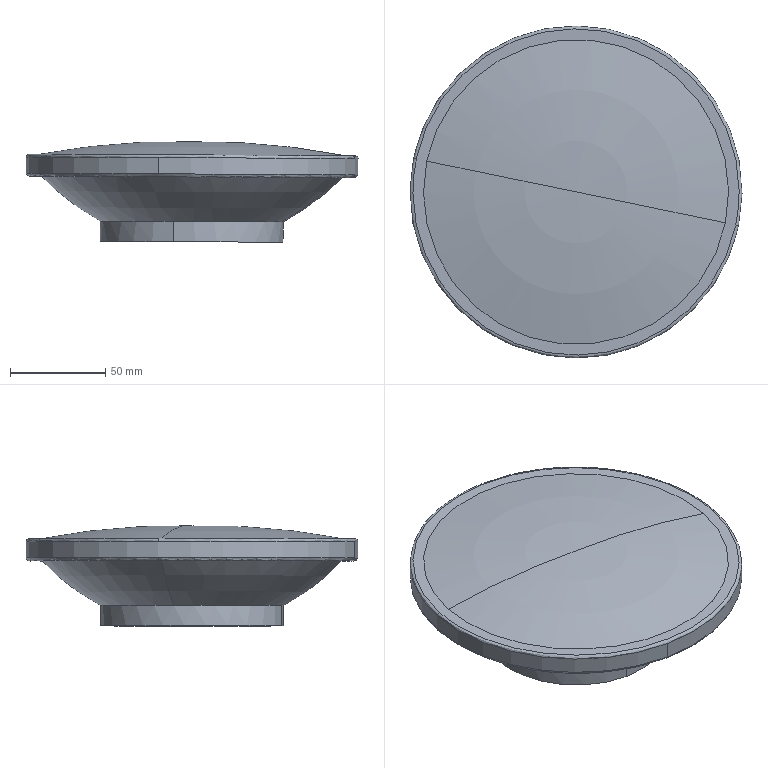Component | SolidWorks | Light-1_YellowLight-1 | 1 solid | 15 faces | box 174.03 x 174 x 52.73 mm | volume 739684 mm3 | cylinder 4 | torus 4 | spline 4 | plane 3 | commonest cylinder face diameters 96.01 x2 174 x2
STEP:
#1=COLOUR_RGB('',0.7922,0.8196,0.9333);
#2=FILL_AREA_STYLE_COLOUR('',#1);
#3=FILL_AREA_STYLE('',(#2));
#4=SURFACE_STYLE_FILL_AREA(#3);
#5=SURFACE_SIDE_STYLE('',(#4));
#6=SURFACE_STYLE_USAGE(.BOTH.,#5);
#7=PRESENTATION_STYLE_ASSIGNMENT((#6));
#8=CARTESIAN_POINT('',(-212.011,277.56,12.301));
#9=VERTEX_POINT('',#8);
#10=CARTESIAN_POINT('',(-212.776,273.859,12.304));
#11=VERTEX_POINT('',#10);
#12=CARTESIAN_POINT('',(-212.394,275.71,12.303));
#13=DIRECTION('',(-0.004294,-0.,-1.));
#14=DIRECTION('',(-0.2024,-0.9793,0.0008691));
#15=AXIS2_PLACEMENT_3D('',#12,#13,#14);
#16=CIRCLE('',#15,1.89);
#17=EDGE_CURVE('',#9,#11,#16,.T.);
#18=ORIENTED_EDGE('',*,*,#17,.F.);
#19=CARTESIAN_POINT('',(-212.009,277.56,12.72));
#20=VERTEX_POINT('',#19);
#21=CARTESIAN_POINT('',(-212.011,277.56,12.301));
#22=DIRECTION('',(0.004294,0.,1.));
#23=VECTOR('',#22,39.37);
#24=LINE('',#21,#23);
#25=EDGE_CURVE('',#9,#20,#24,.T.);
#26=ORIENTED_EDGE('',*,*,#25,.T.);
#27=CARTESIAN_POINT('',(-210.541,275.327,12.714));
#28=VERTEX_POINT('',#27);
#29=CARTESIAN_POINT('',(-212.392,275.71,12.722));
#30=DIRECTION('',(0.004294,0.,1.));
#31=DIRECTION('',(-0.9793,0.2024,0.004205));
#32=AXIS2_PLACEMENT_3D('',#29,#30,#31);
#33=CIRCLE('',#32,1.89);
#34=EDGE_CURVE('',#28,#20,#33,.T.);
#35=ORIENTED_EDGE('',*,*,#34,.F.);
#36=CARTESIAN_POINT('',(-212.774,273.859,12.724));
#37=VERTEX_POINT('',#36);
#38=CARTESIAN_POINT('',(-212.392,275.71,12.722));
#39=DIRECTION('',(0.004294,0.,1.));
#40=DIRECTION('',(-0.9793,0.2024,0.004205));
#41=AXIS2_PLACEMENT_3D('',#38,#39,#40);
#42=CIRCLE('',#41,1.89);
#43=EDGE_CURVE('',#37,#28,#42,.T.);
#44=ORIENTED_EDGE('',*,*,#43,.F.);
#45=CARTESIAN_POINT('',(-212.776,273.859,12.304));
#46=DIRECTION('',(0.004294,0.,1.));
#47=VECTOR('',#46,39.37);
#48=LINE('',#45,#47);
#49=EDGE_CURVE('',#11,#37,#48,.T.);
#50=ORIENTED_EDGE('',*,*,#49,.F.);
#51=EDGE_LOOP('',(#18,#26,#35,#44,#50));
#52=FACE_OUTER_BOUND('',#51,.T.);
#53=CARTESIAN_POINT('',(-212.394,275.71,12.303));
#54=DIRECTION('',(0.004294,0.,1.));
#55=DIRECTION('',(-0.2024,-0.9793,0.0008691));
#56=AXIS2_PLACEMENT_3D('',#53,#54,#55);
#57=CYLINDRICAL_SURFACE('',#56,1.89);
#58=ADVANCED_FACE('',(#52),#57,.T.);
#59=CARTESIAN_POINT('',(-214.243,276.092,12.73));
#60=VERTEX_POINT('',#59);
#61=CARTESIAN_POINT('',(-212.392,275.71,12.722));
#62=DIRECTION('',(0.004294,0.,1.));
#63=DIRECTION('',(-0.9793,0.2024,0.004205));
#64=AXIS2_PLACEMENT_3D('',#61,#62,#63);
#65=CIRCLE('',#64,1.89);
#66=EDGE_CURVE('',#60,#37,#65,.T.);
#67=ORIENTED_EDGE('',*,*,#66,.T.);
#68=ORIENTED_EDGE('',*,*,#43,.T.);
#69=CARTESIAN_POINT('',(-209.28,275.067,13.689));
#70=VERTEX_POINT('',#69);
#71=CARTESIAN_POINT('',(-212.982,275.836,17.344));
#72=DIRECTION('',(-0.2024,-0.9793,0.0008691));
#73=DIRECTION('',(0.9793,-0.2024,0.));
#74=AXIS2_PLACEMENT_3D('',#71,#72,#73);
#75=CIRCLE('',#74,5.259);
#76=EDGE_CURVE('',#28,#70,#75,.T.);
#77=ORIENTED_EDGE('',*,*,#76,.T.);
#78=CARTESIAN_POINT('',(-215.495,276.352,13.716));
#79=VERTEX_POINT('',#78);
#80=CARTESIAN_POINT('',(-212.388,275.71,13.702));
#81=DIRECTION('',(-0.004294,-0.,-1.));
#82=DIRECTION('',(-0.9793,0.2024,0.004205));
#83=AXIS2_PLACEMENT_3D('',#80,#81,#82);
#84=CIRCLE('',#83,3.173);
#85=EDGE_CURVE('',#70,#79,#84,.T.);
#86=ORIENTED_EDGE('',*,*,#85,.T.);
#87=CARTESIAN_POINT('',(-211.762,275.583,17.338));
#88=DIRECTION('',(0.2024,0.9793,-0.0008691));
#89=DIRECTION('',(-0.9793,0.2024,0.));
#90=AXIS2_PLACEMENT_3D('',#87,#88,#89);
#91=CIRCLE('',#90,5.259);
#92=EDGE_CURVE('',#60,#79,#91,.T.);
#93=ORIENTED_EDGE('',*,*,#92,.F.);
#94=EDGE_LOOP('',(#67,#68,#77,#86,#93));
#95=FACE_OUTER_BOUND('',#94,.T.);
#96=CARTESIAN_POINT('',(-212.372,275.71,17.341));
#97=DIRECTION('',(0.004294,0.,1.));
#98=DIRECTION('',(-0.9793,0.2024,0.004205));
#99=AXIS2_PLACEMENT_3D('',#96,#97,#98);
#100=TOROIDAL_SURFACE('',#99,-0.6233,5.259);
#101=ADVANCED_FACE('',(#95),#100,.T.);
#102=CARTESIAN_POINT('',(-211.694,279.064,13.699));
#103=VERTEX_POINT('',#102);
#104=CARTESIAN_POINT('',(-209.033,275.016,13.688));
#105=VERTEX_POINT('',#104);
#106=CARTESIAN_POINT('',(-212.388,275.71,13.702));
#107=DIRECTION('',(-0.004294,-0.,-1.));
#108=DIRECTION('',(0.9793,-0.2024,-0.004205));
#109=AXIS2_PLACEMENT_3D('',#106,#107,#108);
#110=CIRCLE('',#109,3.425);
#111=EDGE_CURVE('',#103,#105,#110,.T.);
#112=ORIENTED_EDGE('',*,*,#111,.F.);
#113=CARTESIAN_POINT('',(-211.693,279.064,14.034));
#114=VERTEX_POINT('',#113);
#115=CARTESIAN_POINT('',(-211.694,279.064,13.699));
#116=DIRECTION('',(0.004294,0.,1.));
#117=VECTOR('',#116,39.37);
#118=LINE('',#115,#117);
#119=EDGE_CURVE('',#103,#114,#118,.T.);
#120=ORIENTED_EDGE('',*,*,#119,.T.);
#121=CARTESIAN_POINT('',(-209.032,275.016,14.023));
#122=VERTEX_POINT('',#121);
#123=CARTESIAN_POINT('',(-212.386,275.71,14.037));
#124=DIRECTION('',(0.004294,0.,1.));
#125=DIRECTION('',(-0.9793,0.2024,0.004205));
#126=AXIS2_PLACEMENT_3D('',#123,#124,#125);
#127=CIRCLE('',#126,3.425);
#128=EDGE_CURVE('',#122,#114,#127,.T.);
#129=ORIENTED_EDGE('',*,*,#128,.F.);
#130=CARTESIAN_POINT('',(-213.079,272.355,14.04));
#131=VERTEX_POINT('',#130);
#132=CARTESIAN_POINT('',(-212.386,275.71,14.037));
#133=DIRECTION('',(0.004294,0.,1.));
#134=DIRECTION('',(-0.9793,0.2024,0.004205));
#135=AXIS2_PLACEMENT_3D('',#132,#133,#134);
#136=CIRCLE('',#135,3.425);
#137=EDGE_CURVE('',#131,#122,#136,.T.);
#138=ORIENTED_EDGE('',*,*,#137,.F.);
#139=CARTESIAN_POINT('',(-213.081,272.355,13.705));
#140=VERTEX_POINT('',#139);
#141=CARTESIAN_POINT('',(-213.081,272.355,13.705));
#142=DIRECTION('',(0.004294,0.,1.));
#143=VECTOR('',#142,39.37);
#144=LINE('',#141,#143);
#145=EDGE_CURVE('',#140,#131,#144,.T.);
#146=ORIENTED_EDGE('',*,*,#145,.F.);
#147=CARTESIAN_POINT('',(-212.388,275.71,13.702));
#148=DIRECTION('',(-0.004294,-0.,-1.));
#149=DIRECTION('',(-0.9793,0.2024,0.004205));
#150=AXIS2_PLACEMENT_3D('',#147,#148,#149);
#151=CIRCLE('',#150,3.425);
#152=EDGE_CURVE('',#105,#140,#151,.T.);
#153=ORIENTED_EDGE('',*,*,#152,.F.);
#154=EDGE_LOOP('',(#112,#120,#129,#138,#146,#153));
#155=FACE_OUTER_BOUND('',#154,.T.);
#156=CARTESIAN_POINT('',(-212.388,275.71,13.702));
#157=DIRECTION('',(0.004294,0.,1.));
#158=DIRECTION('',(-0.2024,-0.9793,0.0008691));
#159=AXIS2_PLACEMENT_3D('',#156,#157,#158);
#160=CYLINDRICAL_SURFACE('',#159,3.425);
#161=ADVANCED_FACE('',(#155),#160,.T.);
#162=CARTESIAN_POINT('',(-209.303,275.072,14.083));
#163=VERTEX_POINT('',#162);
#164=CARTESIAN_POINT('',(-215.469,276.347,14.109));
#165=VERTEX_POINT('',#164);
#166=CARTESIAN_POINT('',(-212.386,275.71,14.096));
#167=DIRECTION('',(-0.004294,-0.,-1.));
#168=DIRECTION('',(-0.9793,0.2024,0.004205));
#169=AXIS2_PLACEMENT_3D('',#166,#167,#168);
#170=CIRCLE('',#169,3.148);
#171=EDGE_CURVE('',#163,#165,#170,.T.);
#172=ORIENTED_EDGE('',*,*,#171,.F.);
#173=CARTESIAN_POINT('',(-212.385,275.71,14.366));
#174=VERTEX_POINT('',#173);
#175=CARTESIAN_POINT('',(-212.166,275.651,-0.7306));
#176=DIRECTION('',(-0.2024,-0.9793,0.0008691));
#177=DIRECTION('',(0.9793,-0.2024,0.));
#178=AXIS2_PLACEMENT_3D('',#175,#176,#177);
#179=CIRCLE('',#178,15.099);
#180=EDGE_CURVE('',#163,#174,#179,.T.);
#181=ORIENTED_EDGE('',*,*,#180,.T.);
#182=CARTESIAN_POINT('',(-212.733,275.768,-0.7281));
#183=DIRECTION('',(0.2024,0.9793,-0.0008691));
#184=DIRECTION('',(-0.9793,0.2024,0.));
#185=AXIS2_PLACEMENT_3D('',#182,#183,#184);
#186=CIRCLE('',#185,15.099);
#187=EDGE_CURVE('',#165,#174,#186,.T.);
#188=ORIENTED_EDGE('',*,*,#187,.F.);
#189=EDGE_LOOP('',(#172,#181,#188));
#190=FACE_OUTER_BOUND('',#189,.T.);
#191=CARTESIAN_POINT('',(-212.45,275.71,-0.7293));
#192=DIRECTION('',(0.004294,0.,1.));
#193=DIRECTION('',(-0.9793,0.2024,0.004205));
#194=AXIS2_PLACEMENT_3D('',#191,#192,#193);
#195=TOROIDAL_SURFACE('',#194,0.2891,15.099);
#196=ADVANCED_FACE('',(#190),#195,.T.);
#197=ORIENTED_EDGE('',*,*,#25,.F.);
#198=CARTESIAN_POINT('',(-212.394,275.71,12.303));
#199=DIRECTION('',(-0.004294,-0.,-1.));
#200=DIRECTION('',(-0.2024,-0.9793,0.0008691));
#201=AXIS2_PLACEMENT_3D('',#198,#199,#200);
#202=CIRCLE('',#201,1.89);
#203=EDGE_CURVE('',#11,#9,#202,.T.);
#204=ORIENTED_EDGE('',*,*,#203,.F.);
#205=ORIENTED_EDGE('',*,*,#49,.T.);
#206=ORIENTED_EDGE('',*,*,#66,.F.);
#207=CARTESIAN_POINT('',(-212.392,275.71,12.722));
#208=DIRECTION('',(0.004294,0.,1.));
#209=DIRECTION('',(-0.9793,0.2024,0.004205));
#210=AXIS2_PLACEMENT_3D('',#207,#208,#209);
#211=CIRCLE('',#210,1.89);
#212=EDGE_CURVE('',#20,#60,#211,.T.);
#213=ORIENTED_EDGE('',*,*,#212,.F.);
#214=EDGE_LOOP('',(#197,#204,#205,#206,#213));
#215=FACE_OUTER_BOUND('',#214,.T.);
#216=CARTESIAN_POINT('',(-212.394,275.71,12.303));
#217=DIRECTION('',(0.004294,0.,1.));
#218=DIRECTION('',(-0.2024,-0.9793,0.0008691));
#219=AXIS2_PLACEMENT_3D('',#216,#217,#218);
#220=CYLINDRICAL_SURFACE('',#219,1.89);
#221=ADVANCED_FACE('',(#215),#220,.T.);
#222=ORIENTED_EDGE('',*,*,#203,.T.);
#223=ORIENTED_EDGE('',*,*,#17,.T.);
#224=EDGE_LOOP('',(#222,#223));
#225=FACE_OUTER_BOUND('',#224,.T.);
#226=CARTESIAN_POINT('',(-213.879,277.97,12.309));
#227=DIRECTION('',(-0.004294,-0.,-1.));
#228=DIRECTION('',(0.9793,-0.2024,-0.004205));
#229=AXIS2_PLACEMENT_3D('',#226,#227,#228);
#230=PLANE('',#229);
#231=ADVANCED_FACE('',(#225),#230,.T.);
#232=ORIENTED_EDGE('',*,*,#76,.F.);
#233=ORIENTED_EDGE('',*,*,#34,.T.);
#234=ORIENTED_EDGE('',*,*,#212,.T.);
#235=ORIENTED_EDGE('',*,*,#92,.T.);
#236=CARTESIAN_POINT('',(-212.388,275.71,13.702));
#237=DIRECTION('',(-0.004294,-0.,-1.));
#238=DIRECTION('',(-0.9793,0.2024,0.004205));
#239=AXIS2_PLACEMENT_3D('',#236,#237,#238);
#240=CIRCLE('',#239,3.173);
#241=EDGE_CURVE('',#79,#70,#240,.T.);
#242=ORIENTED_EDGE('',*,*,#241,.T.);
#243=EDGE_LOOP('',(#232,#233,#234,#235,#242));
#244=FACE_OUTER_BOUND('',#243,.T.);
#245=CARTESIAN_POINT('',(-212.372,275.71,17.341));
#246=DIRECTION('',(0.004294,0.,1.));
#247=DIRECTION('',(-0.9793,0.2024,0.004205));
#248=AXIS2_PLACEMENT_3D('',#245,#246,#247);
#249=TOROIDAL_SURFACE('',#248,-0.6233,5.259);
#250=ADVANCED_FACE('',(#244),#249,.T.);
#251=ORIENTED_EDGE('',*,*,#241,.F.);
#252=ORIENTED_EDGE('',*,*,#85,.F.);
#253=EDGE_LOOP('',(#251,#252));
#254=FACE_BOUND('',#253,.T.);
#255=CARTESIAN_POINT('',(-209.198,275.05,13.689));
#256=VERTEX_POINT('',#255);
#257=CARTESIAN_POINT('',(-215.577,276.369,13.716));
#258=VERTEX_POINT('',#257);
#259=CARTESIAN_POINT('',(-209.198,275.05,13.689));
#260=CARTESIAN_POINT('',(-210.517,268.671,13.694));
#261=CARTESIAN_POINT('',(-216.896,269.99,13.722));
#262=CARTESIAN_POINT('',(-215.577,276.369,13.716));
#263=(BOUNDED_CURVE()B_SPLINE_CURVE(3,(#259,#260,#261,#262),.UNSPECIFIED.,.F.,.F.)B_SPLINE_CURVE_WITH_KNOTS((4,4),(0.,0.2611),.UNSPECIFIED.)CURVE()GEOMETRIC_REPRESENTATION_ITEM()RATIONAL_B_SPLINE_CURVE((0.9227,0.3076,0.3076,0.9227))REPRESENTATION_ITEM(''));
#264=EDGE_CURVE('',#256,#258,#263,.T.);
#265=ORIENTED_EDGE('',*,*,#264,.T.);
#266=CARTESIAN_POINT('',(-215.577,276.369,13.716));
#267=CARTESIAN_POINT('',(-214.259,282.748,13.71));
#268=CARTESIAN_POINT('',(-207.879,281.43,13.683));
#269=CARTESIAN_POINT('',(-209.198,275.05,13.689));
#270=(BOUNDED_CURVE()B_SPLINE_CURVE(3,(#266,#267,#268,#269),.UNSPECIFIED.,.F.,.F.)B_SPLINE_CURVE_WITH_KNOTS((4,4),(0.,0.2611),.UNSPECIFIED.)CURVE()GEOMETRIC_REPRESENTATION_ITEM()RATIONAL_B_SPLINE_CURVE((0.9227,0.3076,0.3076,0.9227))REPRESENTATION_ITEM(''));
#271=EDGE_CURVE('',#258,#256,#270,.T.);
#272=ORIENTED_EDGE('',*,*,#271,.T.);
#273=EDGE_LOOP('',(#265,#272));
#274=FACE_OUTER_BOUND('',#273,.T.);
#275=CARTESIAN_POINT('',(-214.948,279.605,13.713));
#276=DIRECTION('',(-0.004294,-0.,-1.));
#277=DIRECTION('',(0.9793,-0.2024,-0.004205));
#278=AXIS2_PLACEMENT_3D('',#275,#276,#277);
#279=PLANE('',#278);
#280=ADVANCED_FACE('',(#254,#274),#279,.T.);
#281=CARTESIAN_POINT('',(-215.742,276.403,13.717));
#282=VERTEX_POINT('',#281);
#283=CARTESIAN_POINT('',(-215.577,276.369,13.716));
#284=CARTESIAN_POINT('',(-215.606,276.375,13.61));
#285=CARTESIAN_POINT('',(-215.714,276.397,13.61));
#286=CARTESIAN_POINT('',(-215.742,276.403,13.717));
#287=(BOUNDED_CURVE()B_SPLINE_CURVE(3,(#283,#284,#285,#286),.UNSPECIFIED.,.F.,.F.)B_SPLINE_CURVE_WITH_KNOTS((4,4),(0.04868,0.9513),.UNSPECIFIED.)CURVE()GEOMETRIC_REPRESENTATION_ITEM()RATIONAL_B_SPLINE_CURVE((0.9227,0.4691,0.4691,0.9227))REPRESENTATION_ITEM(''));
#288=EDGE_CURVE('',#258,#282,#287,.T.);
#289=ORIENTED_EDGE('',*,*,#288,.T.);
#290=CARTESIAN_POINT('',(-212.388,275.71,13.702));
#291=DIRECTION('',(-0.004294,-0.,-1.));
#292=DIRECTION('',(0.9793,-0.2024,-0.004205));
#293=AXIS2_PLACEMENT_3D('',#290,#291,#292);
#294=CIRCLE('',#293,3.425);
#295=EDGE_CURVE('',#282,#103,#294,.T.);
#296=ORIENTED_EDGE('',*,*,#295,.T.);
#297=ORIENTED_EDGE('',*,*,#111,.T.);
#298=CARTESIAN_POINT('',(-209.033,275.016,13.688));
#299=CARTESIAN_POINT('',(-209.062,275.022,13.582));
#300=CARTESIAN_POINT('',(-209.17,275.044,13.582));
#301=CARTESIAN_POINT('',(-209.198,275.05,13.689));
#302=(BOUNDED_CURVE()B_SPLINE_CURVE(3,(#298,#299,#300,#301),.UNSPECIFIED.,.F.,.T.)B_SPLINE_CURVE_WITH_KNOTS((4,4),(0.04868,0.9513),.UNSPECIFIED.)CURVE()GEOMETRIC_REPRESENTATION_ITEM()RATIONAL_B_SPLINE_CURVE((0.9227,0.4691,0.4691,0.9227))REPRESENTATION_ITEM(''));
#303=EDGE_CURVE('',#105,#256,#302,.T.);
#304=ORIENTED_EDGE('',*,*,#303,.T.);
#305=ORIENTED_EDGE('',*,*,#271,.F.);
#306=EDGE_LOOP('',(#289,#296,#297,#304,#305));
#307=FACE_OUTER_BOUND('',#306,.T.);
#308=CARTESIAN_POINT('',(-209.031,275.016,13.696));
#309=CARTESIAN_POINT('',(-207.644,281.728,13.691));
#310=CARTESIAN_POINT('',(-214.356,283.116,13.719));
#311=CARTESIAN_POINT('',(-215.744,276.403,13.725));
#312=CARTESIAN_POINT('',(-209.053,275.02,13.569));
#313=CARTESIAN_POINT('',(-207.674,281.691,13.563));
#314=CARTESIAN_POINT('',(-214.344,283.069,13.592));
#315=CARTESIAN_POINT('',(-215.723,276.399,13.598));
#316=CARTESIAN_POINT('',(-209.179,275.046,13.57));
#317=CARTESIAN_POINT('',(-207.853,281.464,13.564));
#318=CARTESIAN_POINT('',(-214.27,282.79,13.592));
#319=CARTESIAN_POINT('',(-215.597,276.373,13.597));
#320=CARTESIAN_POINT('',(-209.2,275.051,13.697));
#321=CARTESIAN_POINT('',(-207.882,281.426,13.692));
#322=CARTESIAN_POINT('',(-214.257,282.744,13.719));
#323=CARTESIAN_POINT('',(-215.575,276.369,13.725));
#324=(BOUNDED_SURFACE()B_SPLINE_SURFACE(3,3,((#308,#309,#310,#311),(#312,#313,#314,#315),(#316,#317,#318,#319),(#320,#321,#322,#323)),.UNSPECIFIED.,.F.,.F.,.T.)B_SPLINE_SURFACE_WITH_KNOTS((4,4),(4,4),(0.,1.),(0.,1.),.UNSPECIFIED.)GEOMETRIC_REPRESENTATION_ITEM()RATIONAL_B_SPLINE_SURFACE(((1.,0.3333,0.3333,1.),(0.4434,0.1478,0.1478,0.4434),(0.4434,0.1478,0.1478,0.4434),(1.,0.3333,0.3333,1.)))REPRESENTATION_ITEM('')SURFACE());
#325=ADVANCED_FACE('',(#307),#324,.T.);
#326=ORIENTED_EDGE('',*,*,#152,.T.);
#327=CARTESIAN_POINT('',(-212.388,275.71,13.702));
#328=DIRECTION('',(-0.004294,-0.,-1.));
#329=DIRECTION('',(-0.9793,0.2024,0.004205));
#330=AXIS2_PLACEMENT_3D('',#327,#328,#329);
#331=CIRCLE('',#330,3.425);
#332=EDGE_CURVE('',#140,#282,#331,.T.);
#333=ORIENTED_EDGE('',*,*,#332,.T.);
#334=ORIENTED_EDGE('',*,*,#288,.F.);
#335=ORIENTED_EDGE('',*,*,#264,.F.);
#336=ORIENTED_EDGE('',*,*,#303,.F.);
#337=EDGE_LOOP('',(#326,#333,#334,#335,#336));
#338=FACE_OUTER_BOUND('',#337,.T.);
#339=CARTESIAN_POINT('',(-215.744,276.403,13.725));
#340=CARTESIAN_POINT('',(-217.131,269.691,13.731));
#341=CARTESIAN_POINT('',(-210.419,268.304,13.702));
#342=CARTESIAN_POINT('',(-209.031,275.016,13.696));
#343=CARTESIAN_POINT('',(-215.723,276.399,13.598));
#344=CARTESIAN_POINT('',(-217.102,269.729,13.604));
#345=CARTESIAN_POINT('',(-210.432,268.35,13.575));
#346=CARTESIAN_POINT('',(-209.053,275.02,13.569));
#347=CARTESIAN_POINT('',(-215.597,276.373,13.597));
#348=CARTESIAN_POINT('',(-216.923,269.955,13.603));
#349=CARTESIAN_POINT('',(-210.506,268.629,13.575));
#350=CARTESIAN_POINT('',(-209.179,275.046,13.57));
#351=CARTESIAN_POINT('',(-215.575,276.369,13.725));
#352=CARTESIAN_POINT('',(-216.893,269.993,13.73));
#353=CARTESIAN_POINT('',(-210.518,268.675,13.703));
#354=CARTESIAN_POINT('',(-209.2,275.051,13.697));
#355=(BOUNDED_SURFACE()B_SPLINE_SURFACE(3,3,((#339,#340,#341,#342),(#343,#344,#345,#346),(#347,#348,#349,#350),(#351,#352,#353,#354)),.UNSPECIFIED.,.F.,.F.,.F.)B_SPLINE_SURFACE_WITH_KNOTS((4,4),(4,4),(0.,1.),(0.,1.),.UNSPECIFIED.)GEOMETRIC_REPRESENTATION_ITEM()RATIONAL_B_SPLINE_SURFACE(((1.,0.3333,0.3333,1.),(0.4434,0.1478,0.1478,0.4434),(0.4434,0.1478,0.1478,0.4434),(1.,0.3333,0.3333,1.)))REPRESENTATION_ITEM('')SURFACE());
#356=ADVANCED_FACE('',(#338),#355,.T.);
#357=ORIENTED_EDGE('',*,*,#119,.F.);
#358=ORIENTED_EDGE('',*,*,#295,.F.);
#359=ORIENTED_EDGE('',*,*,#332,.F.);
#360=ORIENTED_EDGE('',*,*,#145,.T.);
#361=CARTESIAN_POINT('',(-215.74,276.403,14.051));
#362=VERTEX_POINT('',#361);
#363=CARTESIAN_POINT('',(-212.386,275.71,14.037));
#364=DIRECTION('',(0.004294,0.,1.));
#365=DIRECTION('',(-0.9793,0.2024,0.004205));
#366=AXIS2_PLACEMENT_3D('',#363,#364,#365);
#367=CIRCLE('',#366,3.425);
#368=EDGE_CURVE('',#362,#131,#367,.T.);
#369=ORIENTED_EDGE('',*,*,#368,.F.);
#370=CARTESIAN_POINT('',(-212.386,275.71,14.037));
#371=DIRECTION('',(0.004294,0.,1.));
#372=DIRECTION('',(-0.9793,0.2024,0.004205));
#373=AXIS2_PLACEMENT_3D('',#370,#371,#372);
#374=CIRCLE('',#373,3.425);
#375=EDGE_CURVE('',#114,#362,#374,.T.);
#376=ORIENTED_EDGE('',*,*,#375,.F.);
#377=EDGE_LOOP('',(#357,#358,#359,#360,#369,#376));
#378=FACE_OUTER_BOUND('',#377,.T.);
#379=CARTESIAN_POINT('',(-212.388,275.71,13.702));
#380=DIRECTION('',(0.004294,0.,1.));
#381=DIRECTION('',(-0.2024,-0.9793,0.0008691));
#382=AXIS2_PLACEMENT_3D('',#379,#380,#381);
#383=CYLINDRICAL_SURFACE('',#382,3.425);
#384=ADVANCED_FACE('',(#378),#383,.T.);
#385=CARTESIAN_POINT('',(-215.682,276.391,14.11));
#386=VERTEX_POINT('',#385);
#387=CARTESIAN_POINT('',(-215.74,276.403,14.051));
#388=CARTESIAN_POINT('',(-215.74,276.403,14.086));
#389=CARTESIAN_POINT('',(-215.716,276.398,14.11));
#390=CARTESIAN_POINT('',(-215.682,276.391,14.11));
#391=(BOUNDED_CURVE()B_SPLINE_CURVE(3,(#387,#388,#389,#390),.UNSPECIFIED.,.F.,.F.)B_SPLINE_CURVE_WITH_KNOTS((4,4),(0.06314,0.9369),.UNSPECIFIED.)CURVE()GEOMETRIC_REPRESENTATION_ITEM()RATIONAL_B_SPLINE_CURVE((0.9566,0.7698,0.7698,0.9566))REPRESENTATION_ITEM(''));
#392=EDGE_CURVE('',#362,#386,#391,.T.);
#393=ORIENTED_EDGE('',*,*,#392,.T.);
#394=CARTESIAN_POINT('',(-209.089,275.028,14.082));
#395=VERTEX_POINT('',#394);
#396=CARTESIAN_POINT('',(-215.682,276.391,14.11));
#397=CARTESIAN_POINT('',(-214.32,282.984,14.104));
#398=CARTESIAN_POINT('',(-207.727,281.621,14.076));
#399=CARTESIAN_POINT('',(-209.089,275.028,14.082));
#400=(BOUNDED_CURVE()B_SPLINE_CURVE(3,(#396,#397,#398,#399),.UNSPECIFIED.,.F.,.F.)B_SPLINE_CURVE_WITH_KNOTS((4,4),(0.,1.),.UNSPECIFIED.)CURVE()GEOMETRIC_REPRESENTATION_ITEM()RATIONAL_B_SPLINE_CURVE((0.9566,0.3189,0.3189,0.9566))REPRESENTATION_ITEM(''));
#401=EDGE_CURVE('',#386,#395,#400,.T.);
#402=ORIENTED_EDGE('',*,*,#401,.T.);
#403=CARTESIAN_POINT('',(-209.089,275.028,14.082));
#404=CARTESIAN_POINT('',(-209.056,275.021,14.082));
#405=CARTESIAN_POINT('',(-209.032,275.016,14.057));
#406=CARTESIAN_POINT('',(-209.032,275.016,14.023));
#407=(BOUNDED_CURVE()B_SPLINE_CURVE(3,(#403,#404,#405,#406),.UNSPECIFIED.,.F.,.T.)B_SPLINE_CURVE_WITH_KNOTS((4,4),(0.06314,0.9369),.UNSPECIFIED.)CURVE()GEOMETRIC_REPRESENTATION_ITEM()RATIONAL_B_SPLINE_CURVE((0.9566,0.7698,0.7698,0.9566))REPRESENTATION_ITEM(''));
#408=EDGE_CURVE('',#395,#122,#407,.T.);
#409=ORIENTED_EDGE('',*,*,#408,.T.);
#410=ORIENTED_EDGE('',*,*,#128,.T.);
#411=ORIENTED_EDGE('',*,*,#375,.T.);
#412=EDGE_LOOP('',(#393,#402,#409,#410,#411));
#413=FACE_OUTER_BOUND('',#412,.T.);
#414=CARTESIAN_POINT('',(-209.095,275.029,14.082));
#415=CARTESIAN_POINT('',(-207.735,281.611,14.076));
#416=CARTESIAN_POINT('',(-214.316,282.971,14.104));
#417=CARTESIAN_POINT('',(-215.677,276.39,14.11));
#418=CARTESIAN_POINT('',(-209.056,275.021,14.086));
#419=CARTESIAN_POINT('',(-207.679,281.681,14.08));
#420=CARTESIAN_POINT('',(-214.339,283.058,14.108));
#421=CARTESIAN_POINT('',(-215.716,276.398,14.114));
#422=CARTESIAN_POINT('',(-209.028,275.016,14.057));
#423=CARTESIAN_POINT('',(-207.64,281.731,14.051));
#424=CARTESIAN_POINT('',(-214.356,283.12,14.08));
#425=CARTESIAN_POINT('',(-215.744,276.404,14.086));
#426=CARTESIAN_POINT('',(-209.032,275.016,14.017));
#427=CARTESIAN_POINT('',(-207.646,281.724,14.011));
#428=CARTESIAN_POINT('',(-214.354,283.111,14.04));
#429=CARTESIAN_POINT('',(-215.74,276.403,14.046));
#430=(BOUNDED_SURFACE()B_SPLINE_SURFACE(3,3,((#414,#415,#416,#417),(#418,#419,#420,#421),(#422,#423,#424,#425),(#426,#427,#428,#429)),.UNSPECIFIED.,.F.,.F.,.F.)B_SPLINE_SURFACE_WITH_KNOTS((4,4),(4,4),(0.,1.),(0.,1.),.UNSPECIFIED.)GEOMETRIC_REPRESENTATION_ITEM()RATIONAL_B_SPLINE_SURFACE(((1.,0.3333,0.3333,1.),(0.7553,0.2518,0.2518,0.7553),(0.7553,0.2518,0.2518,0.7553),(1.,0.3333,0.3333,1.)))REPRESENTATION_ITEM('')SURFACE());
#431=ADVANCED_FACE('',(#413),#430,.T.);
#432=CARTESIAN_POINT('',(-209.089,275.028,14.082));
#433=CARTESIAN_POINT('',(-210.452,268.435,14.088));
#434=CARTESIAN_POINT('',(-217.045,269.798,14.116));
#435=CARTESIAN_POINT('',(-215.682,276.391,14.11));
#436=(BOUNDED_CURVE()B_SPLINE_CURVE(3,(#432,#433,#434,#435),.UNSPECIFIED.,.F.,.T.)B_SPLINE_CURVE_WITH_KNOTS((4,4),(0.,1.),.UNSPECIFIED.)CURVE()GEOMETRIC_REPRESENTATION_ITEM()RATIONAL_B_SPLINE_CURVE((0.9566,0.3189,0.3189,0.9566))REPRESENTATION_ITEM(''));
#437=EDGE_CURVE('',#395,#386,#436,.T.);
#438=ORIENTED_EDGE('',*,*,#437,.T.);
#439=ORIENTED_EDGE('',*,*,#392,.F.);
#440=ORIENTED_EDGE('',*,*,#368,.T.);
#441=ORIENTED_EDGE('',*,*,#137,.T.);
#442=ORIENTED_EDGE('',*,*,#408,.F.);
#443=EDGE_LOOP('',(#438,#439,#440,#441,#442));
#444=FACE_OUTER_BOUND('',#443,.T.);
#445=CARTESIAN_POINT('',(-215.677,276.39,14.11));
#446=CARTESIAN_POINT('',(-217.037,269.808,14.116));
#447=CARTESIAN_POINT('',(-210.456,268.448,14.087));
#448=CARTESIAN_POINT('',(-209.095,275.029,14.082));
#449=CARTESIAN_POINT('',(-215.716,276.398,14.114));
#450=CARTESIAN_POINT('',(-217.092,269.738,14.12));
#451=CARTESIAN_POINT('',(-210.433,268.361,14.091));
#452=CARTESIAN_POINT('',(-209.056,275.021,14.086));
#453=CARTESIAN_POINT('',(-215.744,276.404,14.086));
#454=CARTESIAN_POINT('',(-217.132,269.688,14.092));
#455=CARTESIAN_POINT('',(-210.416,268.3,14.063));
#456=CARTESIAN_POINT('',(-209.028,275.016,14.057));
#457=CARTESIAN_POINT('',(-215.74,276.403,14.046));
#458=CARTESIAN_POINT('',(-217.127,269.695,14.051));
#459=CARTESIAN_POINT('',(-210.419,268.308,14.023));
#460=CARTESIAN_POINT('',(-209.032,275.016,14.017));
#461=(BOUNDED_SURFACE()B_SPLINE_SURFACE(3,3,((#445,#446,#447,#448),(#449,#450,#451,#452),(#453,#454,#455,#456),(#457,#458,#459,#460)),.UNSPECIFIED.,.F.,.F.,.F.)B_SPLINE_SURFACE_WITH_KNOTS((4,4),(4,4),(0.,1.),(0.,1.),.UNSPECIFIED.)GEOMETRIC_REPRESENTATION_ITEM()RATIONAL_B_SPLINE_SURFACE(((1.,0.3333,0.3333,1.),(0.7553,0.2518,0.2518,0.7553),(0.7553,0.2518,0.2518,0.7553),(1.,0.3333,0.3333,1.)))REPRESENTATION_ITEM('')SURFACE());
#462=ADVANCED_FACE('',(#444),#461,.T.);
#463=CARTESIAN_POINT('',(-212.386,275.71,14.096));
#464=DIRECTION('',(-0.004294,-0.,-1.));
#465=DIRECTION('',(-0.9793,0.2024,0.004205));
#466=AXIS2_PLACEMENT_3D('',#463,#464,#465);
#467=CIRCLE('',#466,3.148);
#468=EDGE_CURVE('',#165,#163,#467,.T.);
#469=ORIENTED_EDGE('',*,*,#468,.T.);
#470=ORIENTED_EDGE('',*,*,#171,.T.);
#471=EDGE_LOOP('',(#469,#470));
#472=FACE_BOUND('',#471,.T.);
#473=ORIENTED_EDGE('',*,*,#437,.F.);
#474=ORIENTED_EDGE('',*,*,#401,.F.);
#475=EDGE_LOOP('',(#473,#474));
#476=FACE_OUTER_BOUND('',#475,.T.);
#477=CARTESIAN_POINT('',(-208.36,278.356,14.079));
#478=DIRECTION('',(0.004294,0.,1.));
#479=DIRECTION('',(-0.9793,0.2024,0.004205));
#480=AXIS2_PLACEMENT_3D('',#477,#478,#479);
#481=PLANE('',#480);
#482=ADVANCED_FACE('',(#472,#476),#481,.T.);
#483=ORIENTED_EDGE('',*,*,#180,.F.);
#484=ORIENTED_EDGE('',*,*,#468,.F.);
#485=ORIENTED_EDGE('',*,*,#187,.T.);
#486=EDGE_LOOP('',(#483,#484,#485));
#487=FACE_OUTER_BOUND('',#486,.T.);
#488=CARTESIAN_POINT('',(-212.45,275.71,-0.7293));
#489=DIRECTION('',(0.004294,0.,1.));
#490=DIRECTION('',(-0.9793,0.2024,0.004205));
#491=AXIS2_PLACEMENT_3D('',#488,#489,#490);
#492=TOROIDAL_SURFACE('',#491,0.2891,15.099);
#493=ADVANCED_FACE('',(#487),#492,.T.);
#494=CLOSED_SHELL('',(#58,#101,#161,#196,#221,#231,#250,#280,#325,#356,#384,#431,#462,#482,#493));
#495=MANIFOLD_SOLID_BREP('',#494);
#496=STYLED_ITEM('',(#7),#495);
#497=PRESENTATION_LAYER_ASSIGNMENT('','',(#496));
#498=(LENGTH_UNIT()NAMED_UNIT(*)SI_UNIT($,.METRE.));
#499=LENGTH_MEASURE_WITH_UNIT(LENGTH_MEASURE(0.0254),#498);
#500=DIMENSIONAL_EXPONENTS(1.,0.,0.,0.,0.,0.,0.);
#501=(CONVERSION_BASED_UNIT('',#499)LENGTH_UNIT()NAMED_UNIT(#500));
#502=UNCERTAINTY_MEASURE_WITH_UNIT(LENGTH_MEASURE(0.00001),#501,'','');
#503=(NAMED_UNIT(*)PLANE_ANGLE_UNIT()SI_UNIT($,.RADIAN.));
#504=(NAMED_UNIT(*)SI_UNIT($,.STERADIAN.)SOLID_ANGLE_UNIT());
#505=(GEOMETRIC_REPRESENTATION_CONTEXT(3)GLOBAL_UNCERTAINTY_ASSIGNED_CONTEXT((#502))GLOBAL_UNIT_ASSIGNED_CONTEXT((#501,#503,#504))REPRESENTATION_CONTEXT('',''));
#506=MECHANICAL_DESIGN_GEOMETRIC_PRESENTATION_REPRESENTATION('',(#496),#505);
#507=CARTESIAN_POINT('',(0.,0.,0.));
#508=DIRECTION('',(0.,0.,1.));
#509=DIRECTION('',(1.,0.,0.));
#510=AXIS2_PLACEMENT_3D('',#507,#508,#509);
#511=(LENGTH_UNIT()NAMED_UNIT(*)SI_UNIT($,.METRE.));
#512=LENGTH_MEASURE_WITH_UNIT(LENGTH_MEASURE(0.0254),#511);
#513=DIMENSIONAL_EXPONENTS(1.,0.,0.,0.,0.,0.,0.);
#514=(CONVERSION_BASED_UNIT('',#512)LENGTH_UNIT()NAMED_UNIT(#513));
#515=UNCERTAINTY_MEASURE_WITH_UNIT(LENGTH_MEASURE(0.00001),#514,'','');
#516=(NAMED_UNIT(*)PLANE_ANGLE_UNIT()SI_UNIT($,.RADIAN.));
#517=(NAMED_UNIT(*)SI_UNIT($,.STERADIAN.)SOLID_ANGLE_UNIT());
#518=(GEOMETRIC_REPRESENTATION_CONTEXT(3)GLOBAL_UNCERTAINTY_ASSIGNED_CONTEXT((#515))GLOBAL_UNIT_ASSIGNED_CONTEXT((#514,#516,#517))REPRESENTATION_CONTEXT('',''));
#519=ADVANCED_BREP_SHAPE_REPRESENTATION('',(#495,#510),#518);